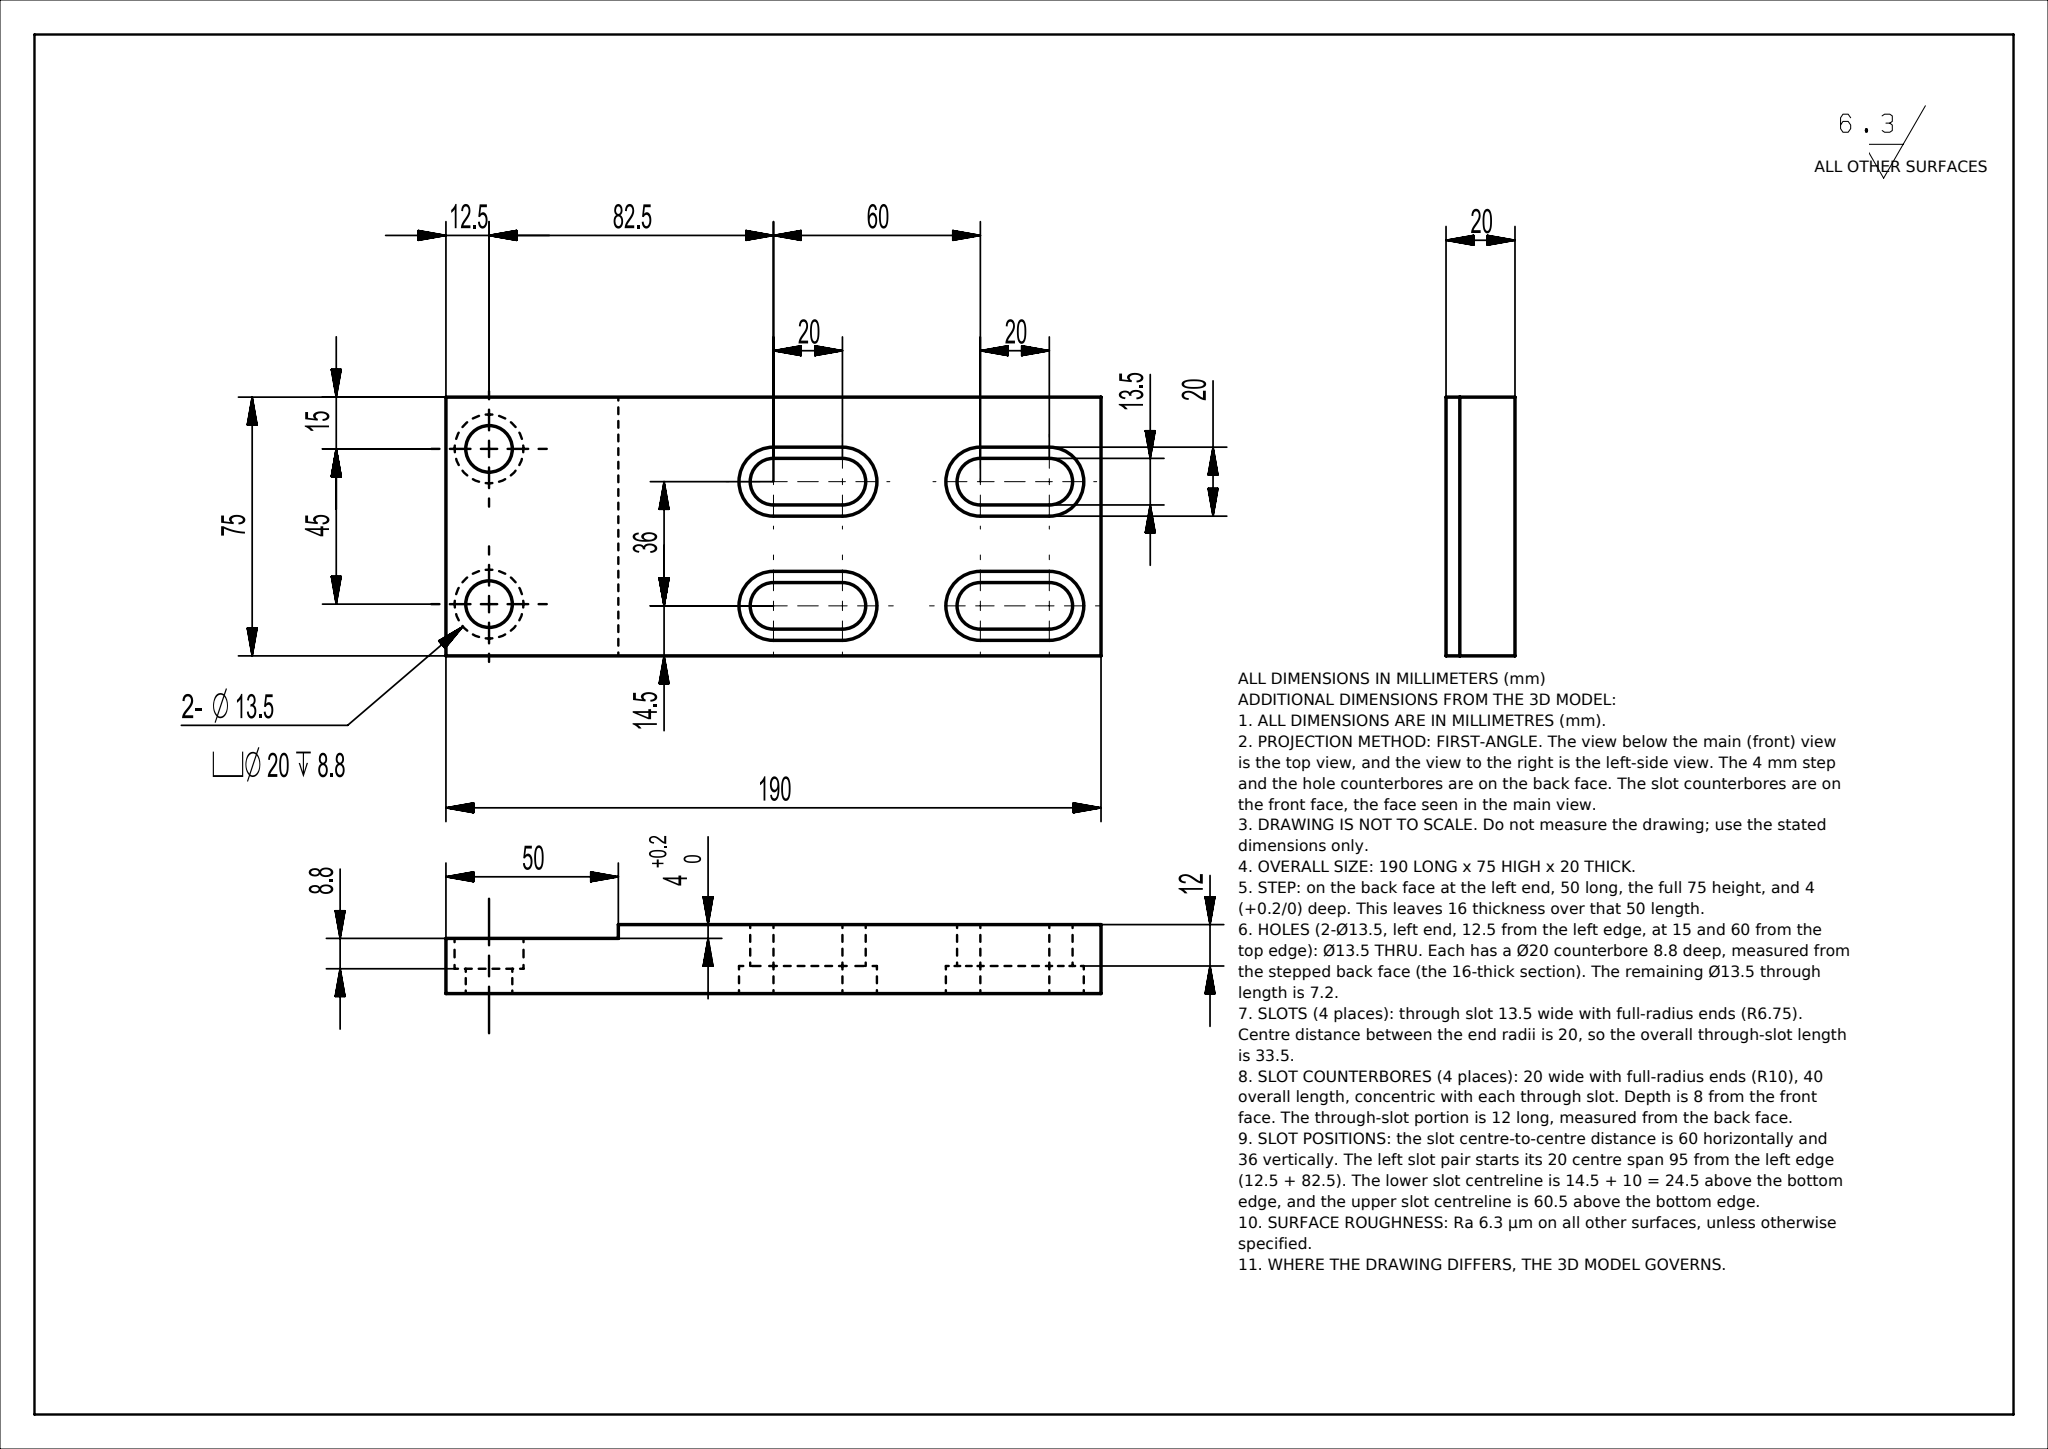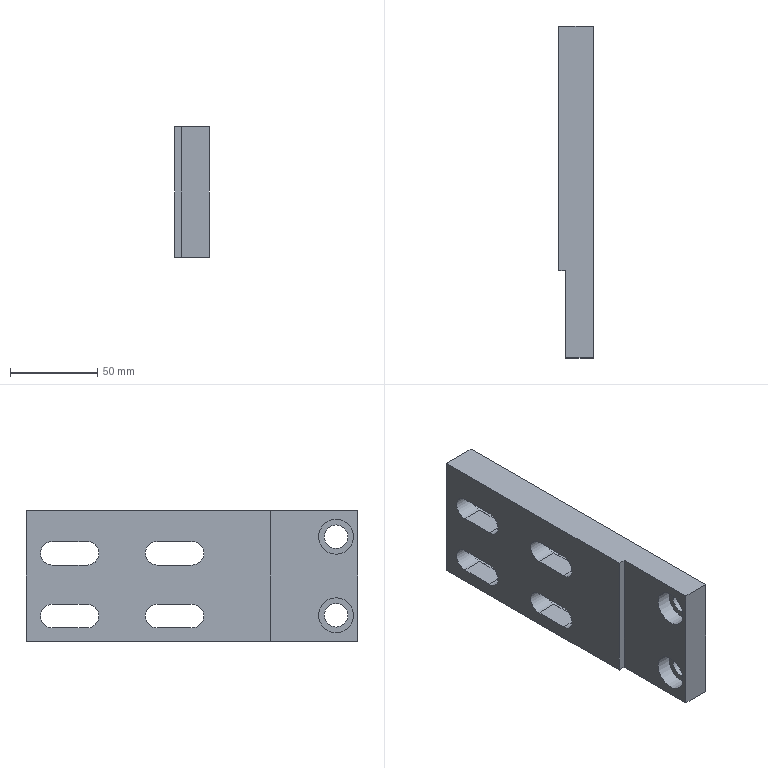Part | NX | mm | 1 solid | 50 faces | box 20 x 190 x 75 mm | volume 219726 mm3 | plane 30 | cylinder 20 | commonest cylinder face diameters 20 x10 13.5 x10